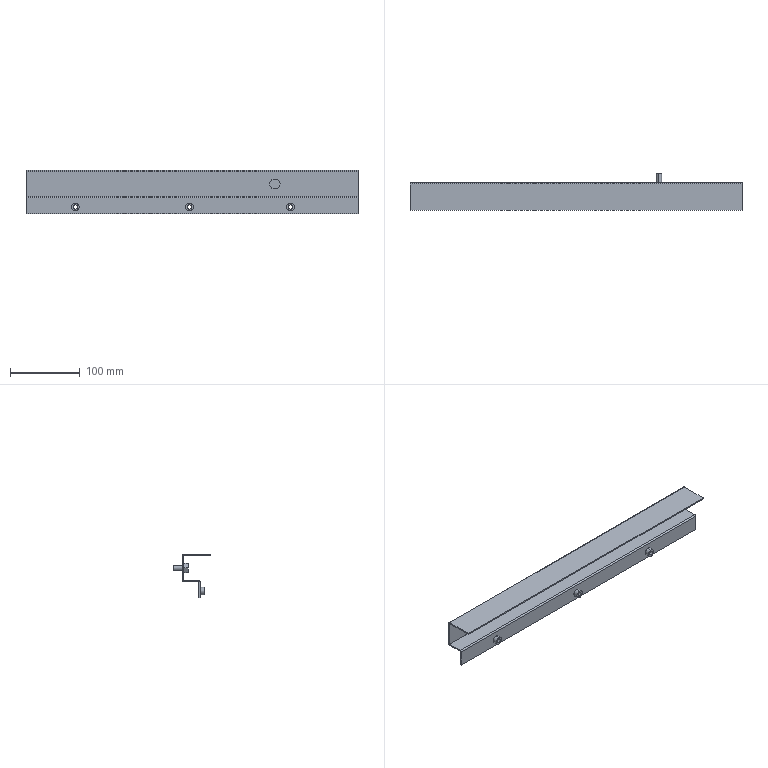Component | SolidWorks | CabinetWelding-1_ShelfSupportBeamRight-1 | 1 solid | 63 faces | volume 108616 mm3 | plane 35 | cylinder 28 | commonest cylinder face diameters 8 x8 6 x6 11 x6 3.8 x3 0.2 x3 7.99 x2